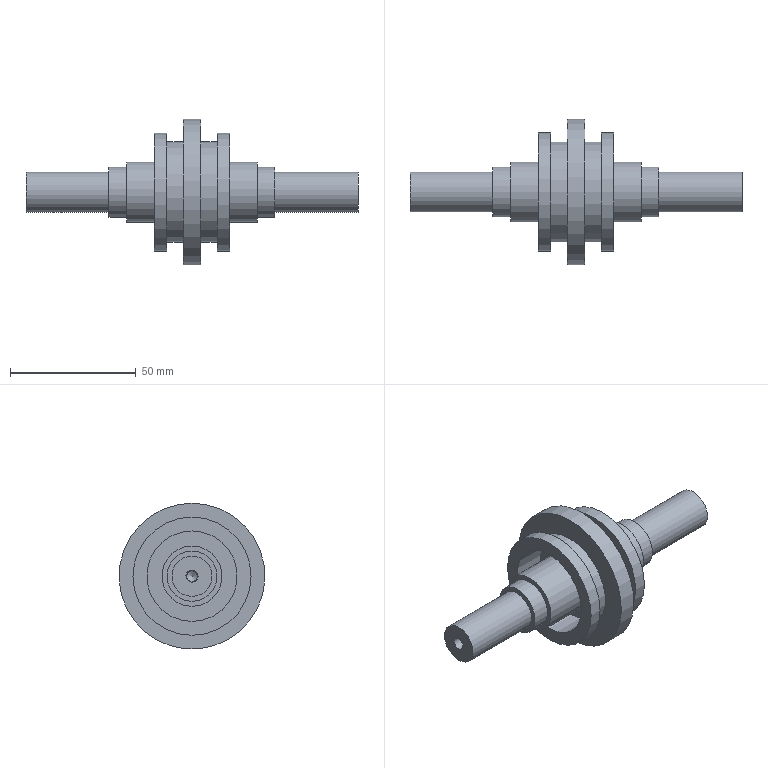Component | NX | FRONT_AXLE | 1 solid | 35 faces | volume 64743 mm3 | cylinder 17 | plane 16 | cone 2 | commonest cylinder face diameters 16 x2 20 x2 24 x2 36 x2 47 x2 40 x2 4.826 x2 4.2 x2